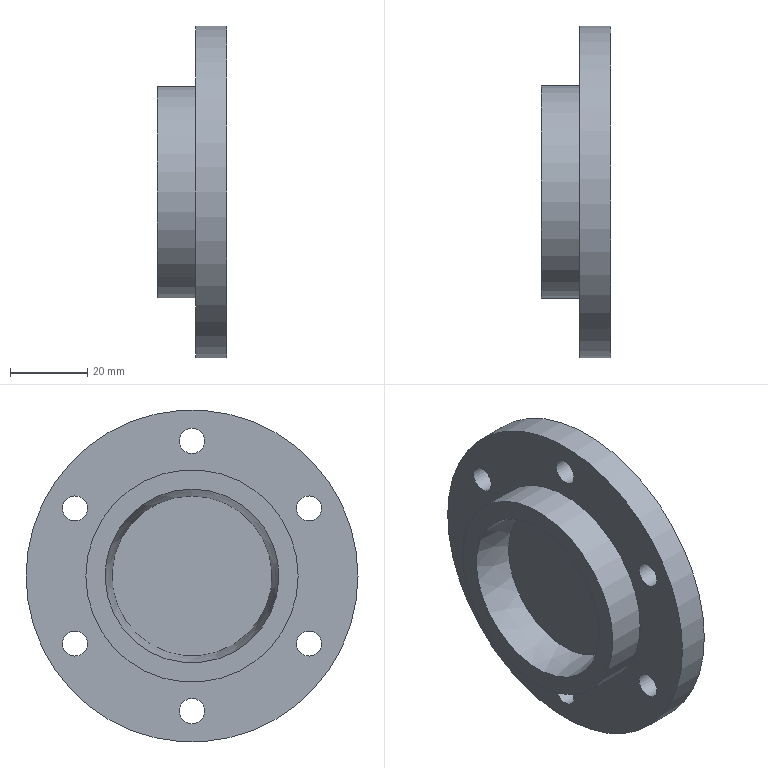Component | NX | XIAODUANMENGAI | 1 solid | 13 faces | box 18 x 86 x 86 mm | volume 53945 mm3 | cylinder 8 | plane 4 | cone 1 | commonest cylinder face diameters 6.5 x6 86 x1 55 x1
STEP:
#1=CARTESIAN_POINT('',(0.,0.,0.));
#2=DIRECTION('',(0.,0.,1.));
#3=DIRECTION('',(1.,0.,0.));
#4=AXIS2_PLACEMENT_3D('',#1,#2,#3);
#5=CARTESIAN_POINT('',(111.,117.811,-73.75));
#6=VERTEX_POINT('',#5);
#7=CARTESIAN_POINT('',(111.,117.811,-67.25));
#8=VERTEX_POINT('',#7);
#9=CARTESIAN_POINT('',(111.,117.811,-70.5));
#10=DIRECTION('',(1.,0.,0.));
#11=DIRECTION('',(0.,0.,-1.));
#12=AXIS2_PLACEMENT_3D('',#9,#10,#11);
#13=CIRCLE('',#12,3.25);
#14=CARTESIAN_POINT('',(111.,87.5,-88.));
#15=DIRECTION('',(1.,0.,0.));
#16=DIRECTION('',(0.,0.,-1.));
#17=AXIS2_PLACEMENT_3D('',#14,#15,#16);
#18=PLANE('',#17);
#19=CARTESIAN_POINT('',(-17.5,30.311));
#20=DIRECTION('',(1.,0.));
#21=AXIS2_PLACEMENT_2D('',#19,#20);
#22=CIRCLE('',#21,3.25);
#23=(GEOMETRIC_REPRESENTATION_CONTEXT(2)PARAMETRIC_REPRESENTATION_CONTEXT()REPRESENTATION_CONTEXT('',''));
#24=DEFINITIONAL_REPRESENTATION('',(#22),#23);
#25=PCURVE('',#18,#24);
#26=CARTESIAN_POINT('',(119.,117.811,-70.5));
#27=DIRECTION('',(-1.,0.,0.));
#28=DIRECTION('',(0.,0.,1.));
#29=AXIS2_PLACEMENT_3D('',#26,#27,#28);
#30=CYLINDRICAL_SURFACE('',#29,3.25);
#31=CARTESIAN_POINT('',(3.142,8.));
#32=DIRECTION('',(-1.,0.));
#33=VECTOR('',#32,1.);
#34=LINE('',#31,#33);
#35=(GEOMETRIC_REPRESENTATION_CONTEXT(2)PARAMETRIC_REPRESENTATION_CONTEXT()REPRESENTATION_CONTEXT('',''));
#36=DEFINITIONAL_REPRESENTATION('',(#34),#35);
#37=PCURVE('',#30,#36);
#38=SURFACE_CURVE('',#13,(#25,#37),.PCURVE_S1.);
#39=EDGE_CURVE('',#6,#8,#38,.T.);
#40=ORIENTED_EDGE('',*,*,#39,.T.);
#41=CARTESIAN_POINT('',(111.,117.811,-70.5));
#42=DIRECTION('',(1.,0.,0.));
#43=DIRECTION('',(0.,0.,-1.));
#44=AXIS2_PLACEMENT_3D('',#41,#42,#43);
#45=CIRCLE('',#44,3.25);
#46=CARTESIAN_POINT('',(-17.5,30.311));
#47=DIRECTION('',(1.,0.));
#48=AXIS2_PLACEMENT_2D('',#46,#47);
#49=CIRCLE('',#48,3.25);
#50=(GEOMETRIC_REPRESENTATION_CONTEXT(2)PARAMETRIC_REPRESENTATION_CONTEXT()REPRESENTATION_CONTEXT('',''));
#51=DEFINITIONAL_REPRESENTATION('',(#49),#50);
#52=PCURVE('',#18,#51);
#53=CARTESIAN_POINT('',(9.425,8.));
#54=DIRECTION('',(-1.,0.));
#55=VECTOR('',#54,1.);
#56=LINE('',#53,#55);
#57=(GEOMETRIC_REPRESENTATION_CONTEXT(2)PARAMETRIC_REPRESENTATION_CONTEXT()REPRESENTATION_CONTEXT('',''));
#58=DEFINITIONAL_REPRESENTATION('',(#56),#57);
#59=PCURVE('',#30,#58);
#60=SURFACE_CURVE('',#45,(#52,#59),.PCURVE_S1.);
#61=EDGE_CURVE('',#8,#6,#60,.T.);
#62=ORIENTED_EDGE('',*,*,#61,.T.);
#63=EDGE_LOOP('',(#40,#62));
#64=FACE_BOUND('',#63,.T.);
#65=CARTESIAN_POINT('',(111.,117.811,-108.75));
#66=VERTEX_POINT('',#65);
#67=CARTESIAN_POINT('',(111.,117.811,-102.25));
#68=VERTEX_POINT('',#67);
#69=CARTESIAN_POINT('',(111.,117.811,-105.5));
#70=DIRECTION('',(1.,0.,0.));
#71=DIRECTION('',(0.,0.,-1.));
#72=AXIS2_PLACEMENT_3D('',#69,#70,#71);
#73=CIRCLE('',#72,3.25);
#74=CARTESIAN_POINT('',(17.5,30.311));
#75=DIRECTION('',(1.,0.));
#76=AXIS2_PLACEMENT_2D('',#74,#75);
#77=CIRCLE('',#76,3.25);
#78=(GEOMETRIC_REPRESENTATION_CONTEXT(2)PARAMETRIC_REPRESENTATION_CONTEXT()REPRESENTATION_CONTEXT('',''));
#79=DEFINITIONAL_REPRESENTATION('',(#77),#78);
#80=PCURVE('',#18,#79);
#81=CARTESIAN_POINT('',(119.,117.811,-105.5));
#82=DIRECTION('',(-1.,0.,0.));
#83=DIRECTION('',(0.,0.,1.));
#84=AXIS2_PLACEMENT_3D('',#81,#82,#83);
#85=CYLINDRICAL_SURFACE('',#84,3.25);
#86=CARTESIAN_POINT('',(3.142,8.));
#87=DIRECTION('',(-1.,0.));
#88=VECTOR('',#87,1.);
#89=LINE('',#86,#88);
#90=(GEOMETRIC_REPRESENTATION_CONTEXT(2)PARAMETRIC_REPRESENTATION_CONTEXT()REPRESENTATION_CONTEXT('',''));
#91=DEFINITIONAL_REPRESENTATION('',(#89),#90);
#92=PCURVE('',#85,#91);
#93=SURFACE_CURVE('',#73,(#80,#92),.PCURVE_S1.);
#94=EDGE_CURVE('',#66,#68,#93,.T.);
#95=ORIENTED_EDGE('',*,*,#94,.T.);
#96=CARTESIAN_POINT('',(111.,117.811,-105.5));
#97=DIRECTION('',(1.,0.,0.));
#98=DIRECTION('',(0.,0.,-1.));
#99=AXIS2_PLACEMENT_3D('',#96,#97,#98);
#100=CIRCLE('',#99,3.25);
#101=CARTESIAN_POINT('',(17.5,30.311));
#102=DIRECTION('',(1.,0.));
#103=AXIS2_PLACEMENT_2D('',#101,#102);
#104=CIRCLE('',#103,3.25);
#105=(GEOMETRIC_REPRESENTATION_CONTEXT(2)PARAMETRIC_REPRESENTATION_CONTEXT()REPRESENTATION_CONTEXT('',''));
#106=DEFINITIONAL_REPRESENTATION('',(#104),#105);
#107=PCURVE('',#18,#106);
#108=CARTESIAN_POINT('',(9.425,8.));
#109=DIRECTION('',(-1.,0.));
#110=VECTOR('',#109,1.);
#111=LINE('',#108,#110);
#112=(GEOMETRIC_REPRESENTATION_CONTEXT(2)PARAMETRIC_REPRESENTATION_CONTEXT()REPRESENTATION_CONTEXT('',''));
#113=DEFINITIONAL_REPRESENTATION('',(#111),#112);
#114=PCURVE('',#85,#113);
#115=SURFACE_CURVE('',#100,(#107,#114),.PCURVE_S1.);
#116=EDGE_CURVE('',#68,#66,#115,.T.);
#117=ORIENTED_EDGE('',*,*,#116,.T.);
#118=EDGE_LOOP('',(#95,#117));
#119=FACE_BOUND('',#118,.T.);
#120=CARTESIAN_POINT('',(111.,87.5,-56.25));
#121=VERTEX_POINT('',#120);
#122=CARTESIAN_POINT('',(111.,87.5,-49.75));
#123=VERTEX_POINT('',#122);
#124=CARTESIAN_POINT('',(111.,87.5,-53.));
#125=DIRECTION('',(1.,0.,0.));
#126=DIRECTION('',(0.,0.,-1.));
#127=AXIS2_PLACEMENT_3D('',#124,#125,#126);
#128=CIRCLE('',#127,3.25);
#129=CARTESIAN_POINT('',(-35.,0.));
#130=DIRECTION('',(1.,0.));
#131=AXIS2_PLACEMENT_2D('',#129,#130);
#132=CIRCLE('',#131,3.25);
#133=(GEOMETRIC_REPRESENTATION_CONTEXT(2)PARAMETRIC_REPRESENTATION_CONTEXT()REPRESENTATION_CONTEXT('',''));
#134=DEFINITIONAL_REPRESENTATION('',(#132),#133);
#135=PCURVE('',#18,#134);
#136=CARTESIAN_POINT('',(119.,87.5,-53.));
#137=DIRECTION('',(-1.,0.,0.));
#138=DIRECTION('',(0.,0.,1.));
#139=AXIS2_PLACEMENT_3D('',#136,#137,#138);
#140=CYLINDRICAL_SURFACE('',#139,3.25);
#141=CARTESIAN_POINT('',(3.142,8.));
#142=DIRECTION('',(-1.,0.));
#143=VECTOR('',#142,1.);
#144=LINE('',#141,#143);
#145=(GEOMETRIC_REPRESENTATION_CONTEXT(2)PARAMETRIC_REPRESENTATION_CONTEXT()REPRESENTATION_CONTEXT('',''));
#146=DEFINITIONAL_REPRESENTATION('',(#144),#145);
#147=PCURVE('',#140,#146);
#148=SURFACE_CURVE('',#128,(#135,#147),.PCURVE_S1.);
#149=EDGE_CURVE('',#121,#123,#148,.T.);
#150=ORIENTED_EDGE('',*,*,#149,.T.);
#151=CARTESIAN_POINT('',(111.,87.5,-53.));
#152=DIRECTION('',(1.,0.,0.));
#153=DIRECTION('',(0.,0.,-1.));
#154=AXIS2_PLACEMENT_3D('',#151,#152,#153);
#155=CIRCLE('',#154,3.25);
#156=CARTESIAN_POINT('',(-35.,0.));
#157=DIRECTION('',(1.,0.));
#158=AXIS2_PLACEMENT_2D('',#156,#157);
#159=CIRCLE('',#158,3.25);
#160=(GEOMETRIC_REPRESENTATION_CONTEXT(2)PARAMETRIC_REPRESENTATION_CONTEXT()REPRESENTATION_CONTEXT('',''));
#161=DEFINITIONAL_REPRESENTATION('',(#159),#160);
#162=PCURVE('',#18,#161);
#163=CARTESIAN_POINT('',(9.425,8.));
#164=DIRECTION('',(-1.,0.));
#165=VECTOR('',#164,1.);
#166=LINE('',#163,#165);
#167=(GEOMETRIC_REPRESENTATION_CONTEXT(2)PARAMETRIC_REPRESENTATION_CONTEXT()REPRESENTATION_CONTEXT('',''));
#168=DEFINITIONAL_REPRESENTATION('',(#166),#167);
#169=PCURVE('',#140,#168);
#170=SURFACE_CURVE('',#155,(#162,#169),.PCURVE_S1.);
#171=EDGE_CURVE('',#123,#121,#170,.T.);
#172=ORIENTED_EDGE('',*,*,#171,.T.);
#173=EDGE_LOOP('',(#150,#172));
#174=FACE_BOUND('',#173,.T.);
#175=CARTESIAN_POINT('',(111.,87.5,-126.25));
#176=VERTEX_POINT('',#175);
#177=CARTESIAN_POINT('',(111.,87.5,-119.75));
#178=VERTEX_POINT('',#177);
#179=CARTESIAN_POINT('',(111.,87.5,-123.));
#180=DIRECTION('',(1.,0.,0.));
#181=DIRECTION('',(0.,0.,-1.));
#182=AXIS2_PLACEMENT_3D('',#179,#180,#181);
#183=CIRCLE('',#182,3.25);
#184=CARTESIAN_POINT('',(35.,0.));
#185=DIRECTION('',(1.,0.));
#186=AXIS2_PLACEMENT_2D('',#184,#185);
#187=CIRCLE('',#186,3.25);
#188=(GEOMETRIC_REPRESENTATION_CONTEXT(2)PARAMETRIC_REPRESENTATION_CONTEXT()REPRESENTATION_CONTEXT('',''));
#189=DEFINITIONAL_REPRESENTATION('',(#187),#188);
#190=PCURVE('',#18,#189);
#191=CARTESIAN_POINT('',(119.,87.5,-123.));
#192=DIRECTION('',(-1.,0.,0.));
#193=DIRECTION('',(0.,0.,1.));
#194=AXIS2_PLACEMENT_3D('',#191,#192,#193);
#195=CYLINDRICAL_SURFACE('',#194,3.25);
#196=CARTESIAN_POINT('',(3.142,8.));
#197=DIRECTION('',(-1.,0.));
#198=VECTOR('',#197,1.);
#199=LINE('',#196,#198);
#200=(GEOMETRIC_REPRESENTATION_CONTEXT(2)PARAMETRIC_REPRESENTATION_CONTEXT()REPRESENTATION_CONTEXT('',''));
#201=DEFINITIONAL_REPRESENTATION('',(#199),#200);
#202=PCURVE('',#195,#201);
#203=SURFACE_CURVE('',#183,(#190,#202),.PCURVE_S1.);
#204=EDGE_CURVE('',#176,#178,#203,.T.);
#205=ORIENTED_EDGE('',*,*,#204,.T.);
#206=CARTESIAN_POINT('',(111.,87.5,-123.));
#207=DIRECTION('',(1.,0.,0.));
#208=DIRECTION('',(0.,0.,-1.));
#209=AXIS2_PLACEMENT_3D('',#206,#207,#208);
#210=CIRCLE('',#209,3.25);
#211=CARTESIAN_POINT('',(35.,0.));
#212=DIRECTION('',(1.,0.));
#213=AXIS2_PLACEMENT_2D('',#211,#212);
#214=CIRCLE('',#213,3.25);
#215=(GEOMETRIC_REPRESENTATION_CONTEXT(2)PARAMETRIC_REPRESENTATION_CONTEXT()REPRESENTATION_CONTEXT('',''));
#216=DEFINITIONAL_REPRESENTATION('',(#214),#215);
#217=PCURVE('',#18,#216);
#218=CARTESIAN_POINT('',(9.425,8.));
#219=DIRECTION('',(-1.,0.));
#220=VECTOR('',#219,1.);
#221=LINE('',#218,#220);
#222=(GEOMETRIC_REPRESENTATION_CONTEXT(2)PARAMETRIC_REPRESENTATION_CONTEXT()REPRESENTATION_CONTEXT('',''));
#223=DEFINITIONAL_REPRESENTATION('',(#221),#222);
#224=PCURVE('',#195,#223);
#225=SURFACE_CURVE('',#210,(#217,#224),.PCURVE_S1.);
#226=EDGE_CURVE('',#178,#176,#225,.T.);
#227=ORIENTED_EDGE('',*,*,#226,.T.);
#228=EDGE_LOOP('',(#205,#227));
#229=FACE_BOUND('',#228,.T.);
#230=CARTESIAN_POINT('',(111.,57.189,-73.75));
#231=VERTEX_POINT('',#230);
#232=CARTESIAN_POINT('',(111.,57.189,-67.25));
#233=VERTEX_POINT('',#232);
#234=CARTESIAN_POINT('',(111.,57.189,-70.5));
#235=DIRECTION('',(1.,0.,0.));
#236=DIRECTION('',(0.,0.,-1.));
#237=AXIS2_PLACEMENT_3D('',#234,#235,#236);
#238=CIRCLE('',#237,3.25);
#239=CARTESIAN_POINT('',(-17.5,-30.311));
#240=DIRECTION('',(1.,0.));
#241=AXIS2_PLACEMENT_2D('',#239,#240);
#242=CIRCLE('',#241,3.25);
#243=(GEOMETRIC_REPRESENTATION_CONTEXT(2)PARAMETRIC_REPRESENTATION_CONTEXT()REPRESENTATION_CONTEXT('',''));
#244=DEFINITIONAL_REPRESENTATION('',(#242),#243);
#245=PCURVE('',#18,#244);
#246=CARTESIAN_POINT('',(119.,57.189,-70.5));
#247=DIRECTION('',(-1.,0.,0.));
#248=DIRECTION('',(0.,0.,1.));
#249=AXIS2_PLACEMENT_3D('',#246,#247,#248);
#250=CYLINDRICAL_SURFACE('',#249,3.25);
#251=CARTESIAN_POINT('',(3.142,8.));
#252=DIRECTION('',(-1.,0.));
#253=VECTOR('',#252,1.);
#254=LINE('',#251,#253);
#255=(GEOMETRIC_REPRESENTATION_CONTEXT(2)PARAMETRIC_REPRESENTATION_CONTEXT()REPRESENTATION_CONTEXT('',''));
#256=DEFINITIONAL_REPRESENTATION('',(#254),#255);
#257=PCURVE('',#250,#256);
#258=SURFACE_CURVE('',#238,(#245,#257),.PCURVE_S1.);
#259=EDGE_CURVE('',#231,#233,#258,.T.);
#260=ORIENTED_EDGE('',*,*,#259,.T.);
#261=CARTESIAN_POINT('',(111.,57.189,-70.5));
#262=DIRECTION('',(1.,0.,0.));
#263=DIRECTION('',(0.,0.,-1.));
#264=AXIS2_PLACEMENT_3D('',#261,#262,#263);
#265=CIRCLE('',#264,3.25);
#266=CARTESIAN_POINT('',(-17.5,-30.311));
#267=DIRECTION('',(1.,0.));
#268=AXIS2_PLACEMENT_2D('',#266,#267);
#269=CIRCLE('',#268,3.25);
#270=(GEOMETRIC_REPRESENTATION_CONTEXT(2)PARAMETRIC_REPRESENTATION_CONTEXT()REPRESENTATION_CONTEXT('',''));
#271=DEFINITIONAL_REPRESENTATION('',(#269),#270);
#272=PCURVE('',#18,#271);
#273=CARTESIAN_POINT('',(9.425,8.));
#274=DIRECTION('',(-1.,0.));
#275=VECTOR('',#274,1.);
#276=LINE('',#273,#275);
#277=(GEOMETRIC_REPRESENTATION_CONTEXT(2)PARAMETRIC_REPRESENTATION_CONTEXT()REPRESENTATION_CONTEXT('',''));
#278=DEFINITIONAL_REPRESENTATION('',(#276),#277);
#279=PCURVE('',#250,#278);
#280=SURFACE_CURVE('',#265,(#272,#279),.PCURVE_S1.);
#281=EDGE_CURVE('',#233,#231,#280,.T.);
#282=ORIENTED_EDGE('',*,*,#281,.T.);
#283=EDGE_LOOP('',(#260,#282));
#284=FACE_BOUND('',#283,.T.);
#285=CARTESIAN_POINT('',(111.,57.189,-108.75));
#286=VERTEX_POINT('',#285);
#287=CARTESIAN_POINT('',(111.,57.189,-102.25));
#288=VERTEX_POINT('',#287);
#289=CARTESIAN_POINT('',(111.,57.189,-105.5));
#290=DIRECTION('',(1.,0.,0.));
#291=DIRECTION('',(0.,0.,-1.));
#292=AXIS2_PLACEMENT_3D('',#289,#290,#291);
#293=CIRCLE('',#292,3.25);
#294=CARTESIAN_POINT('',(17.5,-30.311));
#295=DIRECTION('',(1.,0.));
#296=AXIS2_PLACEMENT_2D('',#294,#295);
#297=CIRCLE('',#296,3.25);
#298=(GEOMETRIC_REPRESENTATION_CONTEXT(2)PARAMETRIC_REPRESENTATION_CONTEXT()REPRESENTATION_CONTEXT('',''));
#299=DEFINITIONAL_REPRESENTATION('',(#297),#298);
#300=PCURVE('',#18,#299);
#301=CARTESIAN_POINT('',(119.,57.189,-105.5));
#302=DIRECTION('',(-1.,0.,0.));
#303=DIRECTION('',(0.,0.,1.));
#304=AXIS2_PLACEMENT_3D('',#301,#302,#303);
#305=CYLINDRICAL_SURFACE('',#304,3.25);
#306=CARTESIAN_POINT('',(3.142,8.));
#307=DIRECTION('',(-1.,0.));
#308=VECTOR('',#307,1.);
#309=LINE('',#306,#308);
#310=(GEOMETRIC_REPRESENTATION_CONTEXT(2)PARAMETRIC_REPRESENTATION_CONTEXT()REPRESENTATION_CONTEXT('',''));
#311=DEFINITIONAL_REPRESENTATION('',(#309),#310);
#312=PCURVE('',#305,#311);
#313=SURFACE_CURVE('',#293,(#300,#312),.PCURVE_S1.);
#314=EDGE_CURVE('',#286,#288,#313,.T.);
#315=ORIENTED_EDGE('',*,*,#314,.T.);
#316=CARTESIAN_POINT('',(111.,57.189,-105.5));
#317=DIRECTION('',(1.,0.,0.));
#318=DIRECTION('',(0.,0.,-1.));
#319=AXIS2_PLACEMENT_3D('',#316,#317,#318);
#320=CIRCLE('',#319,3.25);
#321=CARTESIAN_POINT('',(17.5,-30.311));
#322=DIRECTION('',(1.,0.));
#323=AXIS2_PLACEMENT_2D('',#321,#322);
#324=CIRCLE('',#323,3.25);
#325=(GEOMETRIC_REPRESENTATION_CONTEXT(2)PARAMETRIC_REPRESENTATION_CONTEXT()REPRESENTATION_CONTEXT('',''));
#326=DEFINITIONAL_REPRESENTATION('',(#324),#325);
#327=PCURVE('',#18,#326);
#328=CARTESIAN_POINT('',(9.425,8.));
#329=DIRECTION('',(-1.,0.));
#330=VECTOR('',#329,1.);
#331=LINE('',#328,#330);
#332=(GEOMETRIC_REPRESENTATION_CONTEXT(2)PARAMETRIC_REPRESENTATION_CONTEXT()REPRESENTATION_CONTEXT('',''));
#333=DEFINITIONAL_REPRESENTATION('',(#331),#332);
#334=PCURVE('',#305,#333);
#335=SURFACE_CURVE('',#320,(#327,#334),.PCURVE_S1.);
#336=EDGE_CURVE('',#288,#286,#335,.T.);
#337=ORIENTED_EDGE('',*,*,#336,.T.);
#338=EDGE_LOOP('',(#315,#337));
#339=FACE_BOUND('',#338,.T.);
#340=CARTESIAN_POINT('',(111.,130.5,-88.));
#341=VERTEX_POINT('',#340);
#342=CARTESIAN_POINT('',(111.,87.5,-88.));
#343=DIRECTION('',(1.,0.,0.));
#344=DIRECTION('',(0.,1.,0.));
#345=AXIS2_PLACEMENT_3D('',#342,#343,#344);
#346=CIRCLE('',#345,43.);
#347=CARTESIAN_POINT('',(0.,0.));
#348=DIRECTION('',(0.,1.));
#349=AXIS2_PLACEMENT_2D('',#347,#348);
#350=CIRCLE('',#349,43.);
#351=(GEOMETRIC_REPRESENTATION_CONTEXT(2)PARAMETRIC_REPRESENTATION_CONTEXT()REPRESENTATION_CONTEXT('',''));
#352=DEFINITIONAL_REPRESENTATION('',(#350),#351);
#353=PCURVE('',#18,#352);
#354=CARTESIAN_POINT('',(119.,87.5,-88.));
#355=DIRECTION('',(-1.,0.,0.));
#356=DIRECTION('',(0.,0.,1.));
#357=AXIS2_PLACEMENT_3D('',#354,#355,#356);
#358=CYLINDRICAL_SURFACE('',#357,43.);
#359=CARTESIAN_POINT('',(7.854,8.));
#360=DIRECTION('',(-1.,0.));
#361=VECTOR('',#360,1.);
#362=LINE('',#359,#361);
#363=(GEOMETRIC_REPRESENTATION_CONTEXT(2)PARAMETRIC_REPRESENTATION_CONTEXT()REPRESENTATION_CONTEXT('',''));
#364=DEFINITIONAL_REPRESENTATION('',(#362),#363);
#365=PCURVE('',#358,#364);
#366=SURFACE_CURVE('',#346,(#353,#365),.PCURVE_S1.);
#367=EDGE_CURVE('',#341,#341,#366,.T.);
#368=ORIENTED_EDGE('',*,*,#367,.F.);
#369=EDGE_LOOP('',(#368));
#370=FACE_BOUND('',#369,.T.);
#371=CARTESIAN_POINT('',(111.,115.,-88.));
#372=VERTEX_POINT('',#371);
#373=CARTESIAN_POINT('',(111.,87.5,-88.));
#374=DIRECTION('',(-1.,0.,0.));
#375=DIRECTION('',(0.,1.,0.));
#376=AXIS2_PLACEMENT_3D('',#373,#374,#375);
#377=CIRCLE('',#376,27.5);
#378=CARTESIAN_POINT('',(0.,27.5));
#379=CARTESIAN_POINT('',(47.631,27.5));
#380=CARTESIAN_POINT('',(23.816,-13.75));
#381=CARTESIAN_POINT('',(0.,-55.));
#382=CARTESIAN_POINT('',(-23.816,-13.75));
#383=CARTESIAN_POINT('',(-47.631,27.5));
#384=CARTESIAN_POINT('',(0.,27.5));
#385=(BOUNDED_CURVE()B_SPLINE_CURVE(2,(#378,#379,#380,#381,#382,#383,#384),.UNSPECIFIED.,.T.,.F.)B_SPLINE_CURVE_WITH_KNOTS((1,2,2,2,2,1),(-2.094,0.,2.094,4.189,6.283,8.378),.UNSPECIFIED.)CURVE()GEOMETRIC_REPRESENTATION_ITEM()RATIONAL_B_SPLINE_CURVE((1.,0.5,1.,0.5,1.,0.5,1.))REPRESENTATION_ITEM(''));
#386=(GEOMETRIC_REPRESENTATION_CONTEXT(2)PARAMETRIC_REPRESENTATION_CONTEXT()REPRESENTATION_CONTEXT('',''));
#387=DEFINITIONAL_REPRESENTATION('',(#385),#386);
#388=PCURVE('',#18,#387);
#389=CARTESIAN_POINT('',(101.,87.5,-88.));
#390=DIRECTION('',(1.,0.,0.));
#391=DIRECTION('',(0.,0.,-1.));
#392=AXIS2_PLACEMENT_3D('',#389,#390,#391);
#393=CYLINDRICAL_SURFACE('',#392,27.5);
#394=CARTESIAN_POINT('',(7.854,10.));
#395=DIRECTION('',(-1.,0.));
#396=VECTOR('',#395,1.);
#397=LINE('',#394,#396);
#398=(GEOMETRIC_REPRESENTATION_CONTEXT(2)PARAMETRIC_REPRESENTATION_CONTEXT()REPRESENTATION_CONTEXT('',''));
#399=DEFINITIONAL_REPRESENTATION('',(#397),#398);
#400=PCURVE('',#393,#399);
#401=SURFACE_CURVE('',#377,(#388,#400),.PCURVE_S1.);
#402=EDGE_CURVE('',#372,#372,#401,.T.);
#403=ORIENTED_EDGE('',*,*,#402,.F.);
#404=EDGE_LOOP('',(#403));
#405=FACE_BOUND('',#404,.T.);
#406=ADVANCED_FACE('',(#64,#119,#174,#229,#284,#339,#370,#405),#18,.F.);
#407=CARTESIAN_POINT('',(119.,130.5,-88.));
#408=VERTEX_POINT('',#407);
#409=CARTESIAN_POINT('',(119.,87.5,-88.));
#410=DIRECTION('',(1.,0.,0.));
#411=DIRECTION('',(0.,1.,0.));
#412=AXIS2_PLACEMENT_3D('',#409,#410,#411);
#413=CIRCLE('',#412,43.);
#414=CARTESIAN_POINT('',(7.854,0.));
#415=DIRECTION('',(-1.,0.));
#416=VECTOR('',#415,1.);
#417=LINE('',#414,#416);
#418=(GEOMETRIC_REPRESENTATION_CONTEXT(2)PARAMETRIC_REPRESENTATION_CONTEXT()REPRESENTATION_CONTEXT('',''));
#419=DEFINITIONAL_REPRESENTATION('',(#417),#418);
#420=PCURVE('',#358,#419);
#421=CARTESIAN_POINT('',(119.,87.5,-88.));
#422=DIRECTION('',(1.,0.,0.));
#423=DIRECTION('',(0.,0.,-1.));
#424=AXIS2_PLACEMENT_3D('',#421,#422,#423);
#425=PLANE('',#424);
#426=CARTESIAN_POINT('',(0.,0.));
#427=DIRECTION('',(0.,1.));
#428=AXIS2_PLACEMENT_2D('',#426,#427);
#429=CIRCLE('',#428,43.);
#430=(GEOMETRIC_REPRESENTATION_CONTEXT(2)PARAMETRIC_REPRESENTATION_CONTEXT()REPRESENTATION_CONTEXT('',''));
#431=DEFINITIONAL_REPRESENTATION('',(#429),#430);
#432=PCURVE('',#425,#431);
#433=SURFACE_CURVE('',#413,(#420,#432),.PCURVE_S1.);
#434=EDGE_CURVE('',#408,#408,#433,.T.);
#435=ORIENTED_EDGE('',*,*,#434,.F.);
#436=CARTESIAN_POINT('',(119.,130.5,-88.));
#437=CARTESIAN_POINT('',(111.,130.5,-88.));
#438=B_SPLINE_CURVE_WITH_KNOTS('',1,(#436,#437),.UNSPECIFIED.,.F.,.F.,(2,2),(0.,8.),.PIECEWISE_BEZIER_KNOTS.);
#439=CARTESIAN_POINT('',(7.854,0.));
#440=DIRECTION('',(0.,1.));
#441=VECTOR('',#440,1.);
#442=LINE('',#439,#441);
#443=(GEOMETRIC_REPRESENTATION_CONTEXT(2)PARAMETRIC_REPRESENTATION_CONTEXT()REPRESENTATION_CONTEXT('',''));
#444=DEFINITIONAL_REPRESENTATION('',(#442),#443);
#445=PCURVE('',#358,#444);
#446=CARTESIAN_POINT('',(1.571,0.));
#447=DIRECTION('',(0.,1.));
#448=VECTOR('',#447,1.);
#449=LINE('',#446,#448);
#450=(GEOMETRIC_REPRESENTATION_CONTEXT(2)PARAMETRIC_REPRESENTATION_CONTEXT()REPRESENTATION_CONTEXT('',''));
#451=DEFINITIONAL_REPRESENTATION('',(#449),#450);
#452=PCURVE('',#358,#451);
#453=SEAM_CURVE('',#438,(#445,#452),.PCURVE_S1.);
#454=EDGE_CURVE('',#408,#341,#453,.T.);
#455=ORIENTED_EDGE('',*,*,#454,.T.);
#456=ORIENTED_EDGE('',*,*,#367,.T.);
#457=ORIENTED_EDGE('',*,*,#454,.F.);
#458=EDGE_LOOP('',(#435,#455,#456,#457));
#459=FACE_BOUND('',#458,.T.);
#460=ADVANCED_FACE('',(#459),#358,.T.);
#461=CARTESIAN_POINT('',(119.,117.811,-67.25));
#462=VERTEX_POINT('',#461);
#463=CARTESIAN_POINT('',(119.,117.811,-70.5));
#464=DIRECTION('',(-1.,0.,0.));
#465=DIRECTION('',(0.,0.,1.));
#466=AXIS2_PLACEMENT_3D('',#463,#464,#465);
#467=CIRCLE('',#466,3.25);
#468=CARTESIAN_POINT('',(-20.75,30.311));
#469=CARTESIAN_POINT('',(-20.75,35.94));
#470=CARTESIAN_POINT('',(-15.875,33.125));
#471=CARTESIAN_POINT('',(-11.,30.311));
#472=CARTESIAN_POINT('',(-15.875,27.496));
#473=CARTESIAN_POINT('',(-20.75,24.682));
#474=CARTESIAN_POINT('',(-20.75,30.311));
#475=(BOUNDED_CURVE()B_SPLINE_CURVE(2,(#468,#469,#470,#471,#472,#473,#474),.UNSPECIFIED.,.T.,.F.)B_SPLINE_CURVE_WITH_KNOTS((1,2,2,2,2,1),(-2.094,0.,2.094,4.189,6.283,8.378),.UNSPECIFIED.)CURVE()GEOMETRIC_REPRESENTATION_ITEM()RATIONAL_B_SPLINE_CURVE((1.,0.5,1.,0.5,1.,0.5,1.))REPRESENTATION_ITEM(''));
#476=(GEOMETRIC_REPRESENTATION_CONTEXT(2)PARAMETRIC_REPRESENTATION_CONTEXT()REPRESENTATION_CONTEXT('',''));
#477=DEFINITIONAL_REPRESENTATION('',(#475),#476);
#478=PCURVE('',#425,#477);
#479=CARTESIAN_POINT('',(0.,0.));
#480=DIRECTION('',(1.,0.));
#481=VECTOR('',#480,1.);
#482=LINE('',#479,#481);
#483=(GEOMETRIC_REPRESENTATION_CONTEXT(2)PARAMETRIC_REPRESENTATION_CONTEXT()REPRESENTATION_CONTEXT('',''));
#484=DEFINITIONAL_REPRESENTATION('',(#482),#483);
#485=PCURVE('',#30,#484);
#486=SURFACE_CURVE('',#467,(#478,#485),.PCURVE_S1.);
#487=EDGE_CURVE('',#462,#462,#486,.T.);
#488=ORIENTED_EDGE('',*,*,#487,.T.);
#489=EDGE_LOOP('',(#488));
#490=FACE_BOUND('',#489,.T.);
#491=CARTESIAN_POINT('',(119.,117.811,-102.25));
#492=VERTEX_POINT('',#491);
#493=CARTESIAN_POINT('',(119.,117.811,-105.5));
#494=DIRECTION('',(-1.,0.,0.));
#495=DIRECTION('',(0.,0.,1.));
#496=AXIS2_PLACEMENT_3D('',#493,#494,#495);
#497=CIRCLE('',#496,3.25);
#498=CARTESIAN_POINT('',(14.25,30.311));
#499=CARTESIAN_POINT('',(14.25,35.94));
#500=CARTESIAN_POINT('',(19.125,33.125));
#501=CARTESIAN_POINT('',(24.,30.311));
#502=CARTESIAN_POINT('',(19.125,27.496));
#503=CARTESIAN_POINT('',(14.25,24.682));
#504=CARTESIAN_POINT('',(14.25,30.311));
#505=(BOUNDED_CURVE()B_SPLINE_CURVE(2,(#498,#499,#500,#501,#502,#503,#504),.UNSPECIFIED.,.T.,.F.)B_SPLINE_CURVE_WITH_KNOTS((1,2,2,2,2,1),(-2.094,0.,2.094,4.189,6.283,8.378),.UNSPECIFIED.)CURVE()GEOMETRIC_REPRESENTATION_ITEM()RATIONAL_B_SPLINE_CURVE((1.,0.5,1.,0.5,1.,0.5,1.))REPRESENTATION_ITEM(''));
#506=(GEOMETRIC_REPRESENTATION_CONTEXT(2)PARAMETRIC_REPRESENTATION_CONTEXT()REPRESENTATION_CONTEXT('',''));
#507=DEFINITIONAL_REPRESENTATION('',(#505),#506);
#508=PCURVE('',#425,#507);
#509=CARTESIAN_POINT('',(0.,0.));
#510=DIRECTION('',(1.,0.));
#511=VECTOR('',#510,1.);
#512=LINE('',#509,#511);
#513=(GEOMETRIC_REPRESENTATION_CONTEXT(2)PARAMETRIC_REPRESENTATION_CONTEXT()REPRESENTATION_CONTEXT('',''));
#514=DEFINITIONAL_REPRESENTATION('',(#512),#513);
#515=PCURVE('',#85,#514);
#516=SURFACE_CURVE('',#497,(#508,#515),.PCURVE_S1.);
#517=EDGE_CURVE('',#492,#492,#516,.T.);
#518=ORIENTED_EDGE('',*,*,#517,.T.);
#519=EDGE_LOOP('',(#518));
#520=FACE_BOUND('',#519,.T.);
#521=CARTESIAN_POINT('',(119.,87.5,-49.75));
#522=VERTEX_POINT('',#521);
#523=CARTESIAN_POINT('',(119.,87.5,-53.));
#524=DIRECTION('',(-1.,0.,0.));
#525=DIRECTION('',(0.,0.,1.));
#526=AXIS2_PLACEMENT_3D('',#523,#524,#525);
#527=CIRCLE('',#526,3.25);
#528=CARTESIAN_POINT('',(-38.25,0.));
#529=CARTESIAN_POINT('',(-38.25,5.629));
#530=CARTESIAN_POINT('',(-33.375,2.815));
#531=CARTESIAN_POINT('',(-28.5,0.));
#532=CARTESIAN_POINT('',(-33.375,-2.815));
#533=CARTESIAN_POINT('',(-38.25,-5.629));
#534=CARTESIAN_POINT('',(-38.25,0.));
#535=(BOUNDED_CURVE()B_SPLINE_CURVE(2,(#528,#529,#530,#531,#532,#533,#534),.UNSPECIFIED.,.T.,.F.)B_SPLINE_CURVE_WITH_KNOTS((1,2,2,2,2,1),(-2.094,0.,2.094,4.189,6.283,8.378),.UNSPECIFIED.)CURVE()GEOMETRIC_REPRESENTATION_ITEM()RATIONAL_B_SPLINE_CURVE((1.,0.5,1.,0.5,1.,0.5,1.))REPRESENTATION_ITEM(''));
#536=(GEOMETRIC_REPRESENTATION_CONTEXT(2)PARAMETRIC_REPRESENTATION_CONTEXT()REPRESENTATION_CONTEXT('',''));
#537=DEFINITIONAL_REPRESENTATION('',(#535),#536);
#538=PCURVE('',#425,#537);
#539=CARTESIAN_POINT('',(0.,0.));
#540=DIRECTION('',(1.,0.));
#541=VECTOR('',#540,1.);
#542=LINE('',#539,#541);
#543=(GEOMETRIC_REPRESENTATION_CONTEXT(2)PARAMETRIC_REPRESENTATION_CONTEXT()REPRESENTATION_CONTEXT('',''));
#544=DEFINITIONAL_REPRESENTATION('',(#542),#543);
#545=PCURVE('',#140,#544);
#546=SURFACE_CURVE('',#527,(#538,#545),.PCURVE_S1.);
#547=EDGE_CURVE('',#522,#522,#546,.T.);
#548=ORIENTED_EDGE('',*,*,#547,.T.);
#549=EDGE_LOOP('',(#548));
#550=FACE_BOUND('',#549,.T.);
#551=CARTESIAN_POINT('',(119.,87.5,-119.75));
#552=VERTEX_POINT('',#551);
#553=CARTESIAN_POINT('',(119.,87.5,-123.));
#554=DIRECTION('',(-1.,0.,0.));
#555=DIRECTION('',(0.,0.,1.));
#556=AXIS2_PLACEMENT_3D('',#553,#554,#555);
#557=CIRCLE('',#556,3.25);
#558=CARTESIAN_POINT('',(31.75,0.));
#559=CARTESIAN_POINT('',(31.75,5.629));
#560=CARTESIAN_POINT('',(36.625,2.815));
#561=CARTESIAN_POINT('',(41.5,0.));
#562=CARTESIAN_POINT('',(36.625,-2.815));
#563=CARTESIAN_POINT('',(31.75,-5.629));
#564=CARTESIAN_POINT('',(31.75,0.));
#565=(BOUNDED_CURVE()B_SPLINE_CURVE(2,(#558,#559,#560,#561,#562,#563,#564),.UNSPECIFIED.,.T.,.F.)B_SPLINE_CURVE_WITH_KNOTS((1,2,2,2,2,1),(-2.094,0.,2.094,4.189,6.283,8.378),.UNSPECIFIED.)CURVE()GEOMETRIC_REPRESENTATION_ITEM()RATIONAL_B_SPLINE_CURVE((1.,0.5,1.,0.5,1.,0.5,1.))REPRESENTATION_ITEM(''));
#566=(GEOMETRIC_REPRESENTATION_CONTEXT(2)PARAMETRIC_REPRESENTATION_CONTEXT()REPRESENTATION_CONTEXT('',''));
#567=DEFINITIONAL_REPRESENTATION('',(#565),#566);
#568=PCURVE('',#425,#567);
#569=CARTESIAN_POINT('',(0.,0.));
#570=DIRECTION('',(1.,0.));
#571=VECTOR('',#570,1.);
#572=LINE('',#569,#571);
#573=(GEOMETRIC_REPRESENTATION_CONTEXT(2)PARAMETRIC_REPRESENTATION_CONTEXT()REPRESENTATION_CONTEXT('',''));
#574=DEFINITIONAL_REPRESENTATION('',(#572),#573);
#575=PCURVE('',#195,#574);
#576=SURFACE_CURVE('',#557,(#568,#575),.PCURVE_S1.);
#577=EDGE_CURVE('',#552,#552,#576,.T.);
#578=ORIENTED_EDGE('',*,*,#577,.T.);
#579=EDGE_LOOP('',(#578));
#580=FACE_BOUND('',#579,.T.);
#581=CARTESIAN_POINT('',(119.,57.189,-67.25));
#582=VERTEX_POINT('',#581);
#583=CARTESIAN_POINT('',(119.,57.189,-70.5));
#584=DIRECTION('',(-1.,0.,0.));
#585=DIRECTION('',(0.,0.,1.));
#586=AXIS2_PLACEMENT_3D('',#583,#584,#585);
#587=CIRCLE('',#586,3.25);
#588=CARTESIAN_POINT('',(-20.75,-30.311));
#589=CARTESIAN_POINT('',(-20.75,-24.682));
#590=CARTESIAN_POINT('',(-15.875,-27.496));
#591=CARTESIAN_POINT('',(-11.,-30.311));
#592=CARTESIAN_POINT('',(-15.875,-33.125));
#593=CARTESIAN_POINT('',(-20.75,-35.94));
#594=CARTESIAN_POINT('',(-20.75,-30.311));
#595=(BOUNDED_CURVE()B_SPLINE_CURVE(2,(#588,#589,#590,#591,#592,#593,#594),.UNSPECIFIED.,.T.,.F.)B_SPLINE_CURVE_WITH_KNOTS((1,2,2,2,2,1),(-2.094,0.,2.094,4.189,6.283,8.378),.UNSPECIFIED.)CURVE()GEOMETRIC_REPRESENTATION_ITEM()RATIONAL_B_SPLINE_CURVE((1.,0.5,1.,0.5,1.,0.5,1.))REPRESENTATION_ITEM(''));
#596=(GEOMETRIC_REPRESENTATION_CONTEXT(2)PARAMETRIC_REPRESENTATION_CONTEXT()REPRESENTATION_CONTEXT('',''));
#597=DEFINITIONAL_REPRESENTATION('',(#595),#596);
#598=PCURVE('',#425,#597);
#599=CARTESIAN_POINT('',(0.,0.));
#600=DIRECTION('',(1.,0.));
#601=VECTOR('',#600,1.);
#602=LINE('',#599,#601);
#603=(GEOMETRIC_REPRESENTATION_CONTEXT(2)PARAMETRIC_REPRESENTATION_CONTEXT()REPRESENTATION_CONTEXT('',''));
#604=DEFINITIONAL_REPRESENTATION('',(#602),#603);
#605=PCURVE('',#250,#604);
#606=SURFACE_CURVE('',#587,(#598,#605),.PCURVE_S1.);
#607=EDGE_CURVE('',#582,#582,#606,.T.);
#608=ORIENTED_EDGE('',*,*,#607,.T.);
#609=EDGE_LOOP('',(#608));
#610=FACE_BOUND('',#609,.T.);
#611=CARTESIAN_POINT('',(119.,57.189,-102.25));
#612=VERTEX_POINT('',#611);
#613=CARTESIAN_POINT('',(119.,57.189,-105.5));
#614=DIRECTION('',(-1.,0.,0.));
#615=DIRECTION('',(0.,0.,1.));
#616=AXIS2_PLACEMENT_3D('',#613,#614,#615);
#617=CIRCLE('',#616,3.25);
#618=CARTESIAN_POINT('',(14.25,-30.311));
#619=CARTESIAN_POINT('',(14.25,-24.682));
#620=CARTESIAN_POINT('',(19.125,-27.496));
#621=CARTESIAN_POINT('',(24.,-30.311));
#622=CARTESIAN_POINT('',(19.125,-33.125));
#623=CARTESIAN_POINT('',(14.25,-35.94));
#624=CARTESIAN_POINT('',(14.25,-30.311));
#625=(BOUNDED_CURVE()B_SPLINE_CURVE(2,(#618,#619,#620,#621,#622,#623,#624),.UNSPECIFIED.,.T.,.F.)B_SPLINE_CURVE_WITH_KNOTS((1,2,2,2,2,1),(-2.094,0.,2.094,4.189,6.283,8.378),.UNSPECIFIED.)CURVE()GEOMETRIC_REPRESENTATION_ITEM()RATIONAL_B_SPLINE_CURVE((1.,0.5,1.,0.5,1.,0.5,1.))REPRESENTATION_ITEM(''));
#626=(GEOMETRIC_REPRESENTATION_CONTEXT(2)PARAMETRIC_REPRESENTATION_CONTEXT()REPRESENTATION_CONTEXT('',''));
#627=DEFINITIONAL_REPRESENTATION('',(#625),#626);
#628=PCURVE('',#425,#627);
#629=CARTESIAN_POINT('',(0.,0.));
#630=DIRECTION('',(1.,0.));
#631=VECTOR('',#630,1.);
#632=LINE('',#629,#631);
#633=(GEOMETRIC_REPRESENTATION_CONTEXT(2)PARAMETRIC_REPRESENTATION_CONTEXT()REPRESENTATION_CONTEXT('',''));
#634=DEFINITIONAL_REPRESENTATION('',(#632),#633);
#635=PCURVE('',#305,#634);
#636=SURFACE_CURVE('',#617,(#628,#635),.PCURVE_S1.);
#637=EDGE_CURVE('',#612,#612,#636,.T.);
#638=ORIENTED_EDGE('',*,*,#637,.T.);
#639=EDGE_LOOP('',(#638));
#640=FACE_BOUND('',#639,.T.);
#641=ORIENTED_EDGE('',*,*,#434,.T.);
#642=EDGE_LOOP('',(#641));
#643=FACE_BOUND('',#642,.T.);
#644=ADVANCED_FACE('',(#490,#520,#550,#580,#610,#640,#643),#425,.T.);
#645=CARTESIAN_POINT('',(101.,115.,-88.));
#646=VERTEX_POINT('',#645);
#647=CARTESIAN_POINT('',(101.,87.5,-88.));
#648=DIRECTION('',(-1.,0.,0.));
#649=DIRECTION('',(0.,1.,0.));
#650=AXIS2_PLACEMENT_3D('',#647,#648,#649);
#651=CIRCLE('',#650,27.5);
#652=CARTESIAN_POINT('',(7.854,0.));
#653=DIRECTION('',(-1.,0.));
#654=VECTOR('',#653,1.);
#655=LINE('',#652,#654);
#656=(GEOMETRIC_REPRESENTATION_CONTEXT(2)PARAMETRIC_REPRESENTATION_CONTEXT()REPRESENTATION_CONTEXT('',''));
#657=DEFINITIONAL_REPRESENTATION('',(#655),#656);
#658=PCURVE('',#393,#657);
#659=CARTESIAN_POINT('',(101.,87.5,-88.));
#660=DIRECTION('',(-1.,0.,0.));
#661=DIRECTION('',(0.,0.,1.));
#662=AXIS2_PLACEMENT_3D('',#659,#660,#661);
#663=PLANE('',#662);
#664=CARTESIAN_POINT('',(0.,0.));
#665=DIRECTION('',(0.,1.));
#666=AXIS2_PLACEMENT_2D('',#664,#665);
#667=CIRCLE('',#666,27.5);
#668=(GEOMETRIC_REPRESENTATION_CONTEXT(2)PARAMETRIC_REPRESENTATION_CONTEXT()REPRESENTATION_CONTEXT('',''));
#669=DEFINITIONAL_REPRESENTATION('',(#667),#668);
#670=PCURVE('',#663,#669);
#671=SURFACE_CURVE('',#651,(#658,#670),.PCURVE_S1.);
#672=EDGE_CURVE('',#646,#646,#671,.T.);
#673=ORIENTED_EDGE('',*,*,#672,.F.);
#674=CARTESIAN_POINT('',(101.,115.,-88.));
#675=CARTESIAN_POINT('',(111.,115.,-88.));
#676=B_SPLINE_CURVE_WITH_KNOTS('',1,(#674,#675),.UNSPECIFIED.,.F.,.F.,(2,2),(0.,10.),.PIECEWISE_BEZIER_KNOTS.);
#677=CARTESIAN_POINT('',(7.854,0.));
#678=DIRECTION('',(0.,1.));
#679=VECTOR('',#678,1.);
#680=LINE('',#677,#679);
#681=(GEOMETRIC_REPRESENTATION_CONTEXT(2)PARAMETRIC_REPRESENTATION_CONTEXT()REPRESENTATION_CONTEXT('',''));
#682=DEFINITIONAL_REPRESENTATION('',(#680),#681);
#683=PCURVE('',#393,#682);
#684=CARTESIAN_POINT('',(1.571,0.));
#685=DIRECTION('',(0.,1.));
#686=VECTOR('',#685,1.);
#687=LINE('',#684,#686);
#688=(GEOMETRIC_REPRESENTATION_CONTEXT(2)PARAMETRIC_REPRESENTATION_CONTEXT()REPRESENTATION_CONTEXT('',''));
#689=DEFINITIONAL_REPRESENTATION('',(#687),#688);
#690=PCURVE('',#393,#689);
#691=SEAM_CURVE('',#676,(#683,#690),.PCURVE_S1.);
#692=EDGE_CURVE('',#646,#372,#691,.T.);
#693=ORIENTED_EDGE('',*,*,#692,.T.);
#694=ORIENTED_EDGE('',*,*,#402,.T.);
#695=ORIENTED_EDGE('',*,*,#692,.F.);
#696=EDGE_LOOP('',(#673,#693,#694,#695));
#697=FACE_BOUND('',#696,.T.);
#698=ADVANCED_FACE('',(#697),#393,.T.);
#699=CARTESIAN_POINT('',(101.,87.5,-65.5));
#700=VERTEX_POINT('',#699);
#701=CARTESIAN_POINT('',(101.,87.5,-88.));
#702=DIRECTION('',(-1.,0.,0.));
#703=DIRECTION('',(0.,0.,1.));
#704=AXIS2_PLACEMENT_3D('',#701,#702,#703);
#705=CIRCLE('',#704,22.5);
#706=CARTESIAN_POINT('',(0.,0.));
#707=DIRECTION('',(1.,0.));
#708=AXIS2_PLACEMENT_2D('',#706,#707);
#709=CIRCLE('',#708,22.5);
#710=(GEOMETRIC_REPRESENTATION_CONTEXT(2)PARAMETRIC_REPRESENTATION_CONTEXT()REPRESENTATION_CONTEXT('',''));
#711=DEFINITIONAL_REPRESENTATION('',(#709),#710);
#712=PCURVE('',#663,#711);
#713=CARTESIAN_POINT('',(101.,87.5,-88.));
#714=DIRECTION('',(-1.,0.,0.));
#715=DIRECTION('',(0.,0.,1.));
#716=AXIS2_PLACEMENT_3D('',#713,#714,#715);
#717=CONICAL_SURFACE('',#716,22.5,0.1745);
#718=CARTESIAN_POINT('',(0.,0.));
#719=DIRECTION('',(1.,0.));
#720=VECTOR('',#719,1.);
#721=LINE('',#718,#720);
#722=(GEOMETRIC_REPRESENTATION_CONTEXT(2)PARAMETRIC_REPRESENTATION_CONTEXT()REPRESENTATION_CONTEXT('',''));
#723=DEFINITIONAL_REPRESENTATION('',(#721),#722);
#724=PCURVE('',#717,#723);
#725=SURFACE_CURVE('',#705,(#712,#724),.PCURVE_S1.);
#726=EDGE_CURVE('',#700,#700,#725,.T.);
#727=ORIENTED_EDGE('',*,*,#726,.F.);
#728=EDGE_LOOP('',(#727));
#729=FACE_BOUND('',#728,.T.);
#730=ORIENTED_EDGE('',*,*,#672,.T.);
#731=EDGE_LOOP('',(#730));
#732=FACE_BOUND('',#731,.T.);
#733=ADVANCED_FACE('',(#729,#732),#663,.T.);
#734=CARTESIAN_POINT('',(111.,87.5,-67.263));
#735=VERTEX_POINT('',#734);
#736=CARTESIAN_POINT('',(111.,87.5,-88.));
#737=DIRECTION('',(1.,0.,0.));
#738=DIRECTION('',(0.,0.,1.));
#739=AXIS2_PLACEMENT_3D('',#736,#737,#738);
#740=CIRCLE('',#739,20.737);
#741=CARTESIAN_POINT('',(6.283,-10.));
#742=DIRECTION('',(-1.,0.));
#743=VECTOR('',#742,1.);
#744=LINE('',#741,#743);
#745=(GEOMETRIC_REPRESENTATION_CONTEXT(2)PARAMETRIC_REPRESENTATION_CONTEXT()REPRESENTATION_CONTEXT('',''));
#746=DEFINITIONAL_REPRESENTATION('',(#744),#745);
#747=PCURVE('',#717,#746);
#748=CARTESIAN_POINT('',(111.,87.5,-88.));
#749=DIRECTION('',(-1.,0.,0.));
#750=DIRECTION('',(0.,0.,1.));
#751=AXIS2_PLACEMENT_3D('',#748,#749,#750);
#752=PLANE('',#751);
#753=CARTESIAN_POINT('',(20.737,0.));
#754=CARTESIAN_POINT('',(20.737,-35.917));
#755=CARTESIAN_POINT('',(-10.368,-17.959));
#756=CARTESIAN_POINT('',(-41.473,-0.));
#757=CARTESIAN_POINT('',(-10.368,17.959));
#758=CARTESIAN_POINT('',(20.737,35.917));
#759=CARTESIAN_POINT('',(20.737,0.));
#760=(BOUNDED_CURVE()B_SPLINE_CURVE(2,(#753,#754,#755,#756,#757,#758,#759),.UNSPECIFIED.,.T.,.F.)B_SPLINE_CURVE_WITH_KNOTS((1,2,2,2,2,1),(-2.094,0.,2.094,4.189,6.283,8.378),.UNSPECIFIED.)CURVE()GEOMETRIC_REPRESENTATION_ITEM()RATIONAL_B_SPLINE_CURVE((1.,0.5,1.,0.5,1.,0.5,1.))REPRESENTATION_ITEM(''));
#761=(GEOMETRIC_REPRESENTATION_CONTEXT(2)PARAMETRIC_REPRESENTATION_CONTEXT()REPRESENTATION_CONTEXT('',''));
#762=DEFINITIONAL_REPRESENTATION('',(#760),#761);
#763=PCURVE('',#752,#762);
#764=SURFACE_CURVE('',#740,(#747,#763),.PCURVE_S1.);
#765=EDGE_CURVE('',#735,#735,#764,.T.);
#766=ORIENTED_EDGE('',*,*,#765,.F.);
#767=CARTESIAN_POINT('',(111.,87.5,-67.263));
#768=CARTESIAN_POINT('',(101.,87.5,-65.5));
#769=B_SPLINE_CURVE_WITH_KNOTS('',1,(#767,#768),.UNSPECIFIED.,.F.,.F.,(2,2),(-10.154,0.),.PIECEWISE_BEZIER_KNOTS.);
#770=CARTESIAN_POINT('',(6.283,0.));
#771=DIRECTION('',(0.,1.));
#772=VECTOR('',#771,1.);
#773=LINE('',#770,#772);
#774=(GEOMETRIC_REPRESENTATION_CONTEXT(2)PARAMETRIC_REPRESENTATION_CONTEXT()REPRESENTATION_CONTEXT('',''));
#775=DEFINITIONAL_REPRESENTATION('',(#773),#774);
#776=PCURVE('',#717,#775);
#777=CARTESIAN_POINT('',(0.,0.));
#778=DIRECTION('',(0.,1.));
#779=VECTOR('',#778,1.);
#780=LINE('',#777,#779);
#781=(GEOMETRIC_REPRESENTATION_CONTEXT(2)PARAMETRIC_REPRESENTATION_CONTEXT()REPRESENTATION_CONTEXT('',''));
#782=DEFINITIONAL_REPRESENTATION('',(#780),#781);
#783=PCURVE('',#717,#782);
#784=SEAM_CURVE('',#769,(#776,#783),.PCURVE_S1.);
#785=EDGE_CURVE('',#735,#700,#784,.T.);
#786=ORIENTED_EDGE('',*,*,#785,.T.);
#787=ORIENTED_EDGE('',*,*,#726,.F.);
#788=ORIENTED_EDGE('',*,*,#785,.F.);
#789=EDGE_LOOP('',(#766,#786,#787,#788));
#790=FACE_BOUND('',#789,.F.);
#791=ADVANCED_FACE('',(#790),#717,.F.);
#792=ORIENTED_EDGE('',*,*,#765,.F.);
#793=EDGE_LOOP('',(#792));
#794=FACE_BOUND('',#793,.T.);
#795=ADVANCED_FACE('',(#794),#752,.T.);
#796=ORIENTED_EDGE('',*,*,#637,.T.);
#797=CARTESIAN_POINT('',(119.,57.189,-102.25));
#798=CARTESIAN_POINT('',(111.,57.189,-102.25));
#799=B_SPLINE_CURVE_WITH_KNOTS('',1,(#797,#798),.UNSPECIFIED.,.F.,.F.,(2,2),(0.,8.),.PIECEWISE_BEZIER_KNOTS.);
#800=CARTESIAN_POINT('',(6.283,0.));
#801=DIRECTION('',(0.,1.));
#802=VECTOR('',#801,1.);
#803=LINE('',#800,#802);
#804=(GEOMETRIC_REPRESENTATION_CONTEXT(2)PARAMETRIC_REPRESENTATION_CONTEXT()REPRESENTATION_CONTEXT('',''));
#805=DEFINITIONAL_REPRESENTATION('',(#803),#804);
#806=PCURVE('',#305,#805);
#807=CARTESIAN_POINT('',(0.,0.));
#808=DIRECTION('',(0.,1.));
#809=VECTOR('',#808,1.);
#810=LINE('',#807,#809);
#811=(GEOMETRIC_REPRESENTATION_CONTEXT(2)PARAMETRIC_REPRESENTATION_CONTEXT()REPRESENTATION_CONTEXT('',''));
#812=DEFINITIONAL_REPRESENTATION('',(#810),#811);
#813=PCURVE('',#305,#812);
#814=SEAM_CURVE('',#799,(#806,#813),.PCURVE_S1.);
#815=EDGE_CURVE('',#612,#288,#814,.T.);
#816=ORIENTED_EDGE('',*,*,#815,.T.);
#817=ORIENTED_EDGE('',*,*,#336,.T.);
#818=ORIENTED_EDGE('',*,*,#314,.T.);
#819=ORIENTED_EDGE('',*,*,#815,.F.);
#820=EDGE_LOOP('',(#796,#816,#817,#818,#819));
#821=FACE_BOUND('',#820,.F.);
#822=ADVANCED_FACE('',(#821),#305,.F.);
#823=ORIENTED_EDGE('',*,*,#607,.T.);
#824=CARTESIAN_POINT('',(119.,57.189,-67.25));
#825=CARTESIAN_POINT('',(111.,57.189,-67.25));
#826=B_SPLINE_CURVE_WITH_KNOTS('',1,(#824,#825),.UNSPECIFIED.,.F.,.F.,(2,2),(0.,8.),.PIECEWISE_BEZIER_KNOTS.);
#827=CARTESIAN_POINT('',(6.283,0.));
#828=DIRECTION('',(0.,1.));
#829=VECTOR('',#828,1.);
#830=LINE('',#827,#829);
#831=(GEOMETRIC_REPRESENTATION_CONTEXT(2)PARAMETRIC_REPRESENTATION_CONTEXT()REPRESENTATION_CONTEXT('',''));
#832=DEFINITIONAL_REPRESENTATION('',(#830),#831);
#833=PCURVE('',#250,#832);
#834=CARTESIAN_POINT('',(0.,0.));
#835=DIRECTION('',(0.,1.));
#836=VECTOR('',#835,1.);
#837=LINE('',#834,#836);
#838=(GEOMETRIC_REPRESENTATION_CONTEXT(2)PARAMETRIC_REPRESENTATION_CONTEXT()REPRESENTATION_CONTEXT('',''));
#839=DEFINITIONAL_REPRESENTATION('',(#837),#838);
#840=PCURVE('',#250,#839);
#841=SEAM_CURVE('',#826,(#833,#840),.PCURVE_S1.);
#842=EDGE_CURVE('',#582,#233,#841,.T.);
#843=ORIENTED_EDGE('',*,*,#842,.T.);
#844=ORIENTED_EDGE('',*,*,#281,.T.);
#845=ORIENTED_EDGE('',*,*,#259,.T.);
#846=ORIENTED_EDGE('',*,*,#842,.F.);
#847=EDGE_LOOP('',(#823,#843,#844,#845,#846));
#848=FACE_BOUND('',#847,.F.);
#849=ADVANCED_FACE('',(#848),#250,.F.);
#850=ORIENTED_EDGE('',*,*,#577,.T.);
#851=CARTESIAN_POINT('',(119.,87.5,-119.75));
#852=CARTESIAN_POINT('',(111.,87.5,-119.75));
#853=B_SPLINE_CURVE_WITH_KNOTS('',1,(#851,#852),.UNSPECIFIED.,.F.,.F.,(2,2),(0.,8.),.PIECEWISE_BEZIER_KNOTS.);
#854=CARTESIAN_POINT('',(6.283,0.));
#855=DIRECTION('',(0.,1.));
#856=VECTOR('',#855,1.);
#857=LINE('',#854,#856);
#858=(GEOMETRIC_REPRESENTATION_CONTEXT(2)PARAMETRIC_REPRESENTATION_CONTEXT()REPRESENTATION_CONTEXT('',''));
#859=DEFINITIONAL_REPRESENTATION('',(#857),#858);
#860=PCURVE('',#195,#859);
#861=CARTESIAN_POINT('',(0.,0.));
#862=DIRECTION('',(0.,1.));
#863=VECTOR('',#862,1.);
#864=LINE('',#861,#863);
#865=(GEOMETRIC_REPRESENTATION_CONTEXT(2)PARAMETRIC_REPRESENTATION_CONTEXT()REPRESENTATION_CONTEXT('',''));
#866=DEFINITIONAL_REPRESENTATION('',(#864),#865);
#867=PCURVE('',#195,#866);
#868=SEAM_CURVE('',#853,(#860,#867),.PCURVE_S1.);
#869=EDGE_CURVE('',#552,#178,#868,.T.);
#870=ORIENTED_EDGE('',*,*,#869,.T.);
#871=ORIENTED_EDGE('',*,*,#226,.T.);
#872=ORIENTED_EDGE('',*,*,#204,.T.);
#873=ORIENTED_EDGE('',*,*,#869,.F.);
#874=EDGE_LOOP('',(#850,#870,#871,#872,#873));
#875=FACE_BOUND('',#874,.F.);
#876=ADVANCED_FACE('',(#875),#195,.F.);
#877=ORIENTED_EDGE('',*,*,#547,.T.);
#878=CARTESIAN_POINT('',(119.,87.5,-49.75));
#879=CARTESIAN_POINT('',(111.,87.5,-49.75));
#880=B_SPLINE_CURVE_WITH_KNOTS('',1,(#878,#879),.UNSPECIFIED.,.F.,.F.,(2,2),(0.,8.),.PIECEWISE_BEZIER_KNOTS.);
#881=CARTESIAN_POINT('',(6.283,0.));
#882=DIRECTION('',(0.,1.));
#883=VECTOR('',#882,1.);
#884=LINE('',#881,#883);
#885=(GEOMETRIC_REPRESENTATION_CONTEXT(2)PARAMETRIC_REPRESENTATION_CONTEXT()REPRESENTATION_CONTEXT('',''));
#886=DEFINITIONAL_REPRESENTATION('',(#884),#885);
#887=PCURVE('',#140,#886);
#888=CARTESIAN_POINT('',(0.,0.));
#889=DIRECTION('',(0.,1.));
#890=VECTOR('',#889,1.);
#891=LINE('',#888,#890);
#892=(GEOMETRIC_REPRESENTATION_CONTEXT(2)PARAMETRIC_REPRESENTATION_CONTEXT()REPRESENTATION_CONTEXT('',''));
#893=DEFINITIONAL_REPRESENTATION('',(#891),#892);
#894=PCURVE('',#140,#893);
#895=SEAM_CURVE('',#880,(#887,#894),.PCURVE_S1.);
#896=EDGE_CURVE('',#522,#123,#895,.T.);
#897=ORIENTED_EDGE('',*,*,#896,.T.);
#898=ORIENTED_EDGE('',*,*,#171,.T.);
#899=ORIENTED_EDGE('',*,*,#149,.T.);
#900=ORIENTED_EDGE('',*,*,#896,.F.);
#901=EDGE_LOOP('',(#877,#897,#898,#899,#900));
#902=FACE_BOUND('',#901,.F.);
#903=ADVANCED_FACE('',(#902),#140,.F.);
#904=ORIENTED_EDGE('',*,*,#517,.T.);
#905=CARTESIAN_POINT('',(119.,117.811,-102.25));
#906=CARTESIAN_POINT('',(111.,117.811,-102.25));
#907=B_SPLINE_CURVE_WITH_KNOTS('',1,(#905,#906),.UNSPECIFIED.,.F.,.F.,(2,2),(0.,8.),.PIECEWISE_BEZIER_KNOTS.);
#908=CARTESIAN_POINT('',(6.283,0.));
#909=DIRECTION('',(0.,1.));
#910=VECTOR('',#909,1.);
#911=LINE('',#908,#910);
#912=(GEOMETRIC_REPRESENTATION_CONTEXT(2)PARAMETRIC_REPRESENTATION_CONTEXT()REPRESENTATION_CONTEXT('',''));
#913=DEFINITIONAL_REPRESENTATION('',(#911),#912);
#914=PCURVE('',#85,#913);
#915=CARTESIAN_POINT('',(0.,0.));
#916=DIRECTION('',(0.,1.));
#917=VECTOR('',#916,1.);
#918=LINE('',#915,#917);
#919=(GEOMETRIC_REPRESENTATION_CONTEXT(2)PARAMETRIC_REPRESENTATION_CONTEXT()REPRESENTATION_CONTEXT('',''));
#920=DEFINITIONAL_REPRESENTATION('',(#918),#919);
#921=PCURVE('',#85,#920);
#922=SEAM_CURVE('',#907,(#914,#921),.PCURVE_S1.);
#923=EDGE_CURVE('',#492,#68,#922,.T.);
#924=ORIENTED_EDGE('',*,*,#923,.T.);
#925=ORIENTED_EDGE('',*,*,#116,.T.);
#926=ORIENTED_EDGE('',*,*,#94,.T.);
#927=ORIENTED_EDGE('',*,*,#923,.F.);
#928=EDGE_LOOP('',(#904,#924,#925,#926,#927));
#929=FACE_BOUND('',#928,.F.);
#930=ADVANCED_FACE('',(#929),#85,.F.);
#931=ORIENTED_EDGE('',*,*,#487,.T.);
#932=CARTESIAN_POINT('',(119.,117.811,-67.25));
#933=CARTESIAN_POINT('',(111.,117.811,-67.25));
#934=B_SPLINE_CURVE_WITH_KNOTS('',1,(#932,#933),.UNSPECIFIED.,.F.,.F.,(2,2),(0.,8.),.PIECEWISE_BEZIER_KNOTS.);
#935=CARTESIAN_POINT('',(6.283,0.));
#936=DIRECTION('',(0.,1.));
#937=VECTOR('',#936,1.);
#938=LINE('',#935,#937);
#939=(GEOMETRIC_REPRESENTATION_CONTEXT(2)PARAMETRIC_REPRESENTATION_CONTEXT()REPRESENTATION_CONTEXT('',''));
#940=DEFINITIONAL_REPRESENTATION('',(#938),#939);
#941=PCURVE('',#30,#940);
#942=CARTESIAN_POINT('',(0.,0.));
#943=DIRECTION('',(0.,1.));
#944=VECTOR('',#943,1.);
#945=LINE('',#942,#944);
#946=(GEOMETRIC_REPRESENTATION_CONTEXT(2)PARAMETRIC_REPRESENTATION_CONTEXT()REPRESENTATION_CONTEXT('',''));
#947=DEFINITIONAL_REPRESENTATION('',(#945),#946);
#948=PCURVE('',#30,#947);
#949=SEAM_CURVE('',#934,(#941,#948),.PCURVE_S1.);
#950=EDGE_CURVE('',#462,#8,#949,.T.);
#951=ORIENTED_EDGE('',*,*,#950,.T.);
#952=ORIENTED_EDGE('',*,*,#61,.T.);
#953=ORIENTED_EDGE('',*,*,#39,.T.);
#954=ORIENTED_EDGE('',*,*,#950,.F.);
#955=EDGE_LOOP('',(#931,#951,#952,#953,#954));
#956=FACE_BOUND('',#955,.F.);
#957=ADVANCED_FACE('',(#956),#30,.F.);
#958=CLOSED_SHELL('',(#406,#460,#644,#698,#733,#791,#795,#822,#849,#876,#903,#930,#957));
#959=MANIFOLD_SOLID_BREP('',#958);
#960=(LENGTH_UNIT()NAMED_UNIT(*)SI_UNIT(.MILLI.,.METRE.));
#961=UNCERTAINTY_MEASURE_WITH_UNIT(LENGTH_MEASURE(0.000005),#960,'','');
#962=(NAMED_UNIT(*)PLANE_ANGLE_UNIT()SI_UNIT($,.RADIAN.));
#963=(NAMED_UNIT(*)SI_UNIT($,.STERADIAN.)SOLID_ANGLE_UNIT());
#964=(GEOMETRIC_REPRESENTATION_CONTEXT(3)GLOBAL_UNCERTAINTY_ASSIGNED_CONTEXT((#961))GLOBAL_UNIT_ASSIGNED_CONTEXT((#960,#962,#963))REPRESENTATION_CONTEXT('',''));
#965=ADVANCED_BREP_SHAPE_REPRESENTATION('',(#4,#959),#964);